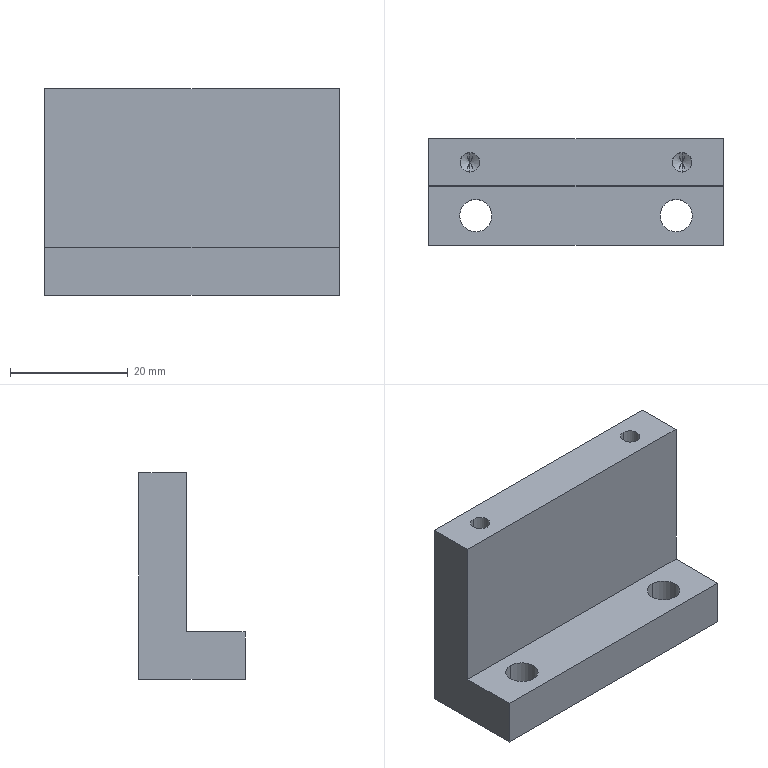Component | SolidWorks | LD101-02--Q1036-Q1-2-2 | 1 solid | 20 faces | box 50 x 18 x 35 mm | volume 17383 mm3 | cylinder 8 | plane 8 | cone 4 | commonest cylinder face diameters 5.5 x4 3.3 x4 | material AL6061
build123d program:
from build123d import *

# Parameters (mm, degrees)
SKETCH1_W             = 50
SKETCH1_H             = 35
BOSS_EXTRUDE1_DEPTH   = 9
SKETCH3_W             = 10
SKETCH3_H             = 27
CUT_EXTRUDE2_DEPTH    = 54.733
M4_TAPPED_HOLE1_D     = 3.3
M4_TAPPED_HOLE1_DEPTH = 13.5
M4_TAPPED_HOLE1_TIP   = 0.9914
SKETCH6_R             = 2.75
CUT_EXTRUDE3_DEPTH    = 38.881


with BuildPart() as part:
    # Sketch1 → Boss-Extrude1 (new, symmetric)
    with BuildSketch(Plane.XY):
        Rectangle(SKETCH1_W, SKETCH1_H)
    extrude(amount=BOSS_EXTRUDE1_DEPTH, both=True)

    # Sketch3 → Cut-Extrude2 (cut, through all)
    with BuildSketch(Plane.ZY.offset(25)):
        with Locations((4, 4)):
            Rectangle(SKETCH3_W, SKETCH3_H)
    extrude(amount=-CUT_EXTRUDE2_DEPTH, mode=Mode.SUBTRACT)

    # M4 Tapped Hole1
    with Locations(Plane(origin=(0, 17.5, 0), x_dir=(1, 0, 0), z_dir=(0, 1, 0))):
        with Locations((-18, 5), (18, 5)):
            Hole(M4_TAPPED_HOLE1_D / 2, depth=M4_TAPPED_HOLE1_DEPTH)
            with Locations((0, 0, -(M4_TAPPED_HOLE1_DEPTH + M4_TAPPED_HOLE1_TIP / 2))):  # 118° drill point
                Cone(0, M4_TAPPED_HOLE1_D / 2, M4_TAPPED_HOLE1_TIP, mode=Mode.SUBTRACT)

    # Sketch6 → Cut-Extrude3 (cut, through all)
    with BuildSketch(Plane(origin=(0, -9.5, 0), x_dir=(1, 0, 0), z_dir=(0, 1, 0))):
        with Locations(Location((-17, -4, 0), (0, 0, 270))):
            Circle(SKETCH6_R)
        with Locations(Location((17, -4, 0), (0, 0, 90))):
            Circle(SKETCH6_R)
    extrude(amount=-CUT_EXTRUDE3_DEPTH, mode=Mode.SUBTRACT)


solid = part.part

# Placed as in the assembly
solid = solid.moved(Location((121.71, -215.897, 310.757), (90, 0, 0)))
STEP:
#1=COLOUR_RGB('',0.7922,0.8196,0.9333);
#2=FILL_AREA_STYLE_COLOUR('',#1);
#3=FILL_AREA_STYLE('',(#2));
#4=SURFACE_STYLE_FILL_AREA(#3);
#5=SURFACE_SIDE_STYLE('',(#4));
#6=SURFACE_STYLE_USAGE(.BOTH.,#5);
#7=PRESENTATION_STYLE_ASSIGNMENT((#6));
#8=CARTESIAN_POINT('',(5.461,-8.549,11.546));
#9=VERTEX_POINT('',#8);
#10=CARTESIAN_POINT('',(5.461,-8.766,11.546));
#11=VERTEX_POINT('',#10);
#12=CARTESIAN_POINT('',(5.461,-8.657,11.546));
#13=DIRECTION('',(-0.,-0.,1.));
#14=DIRECTION('',(0.,1.,0.));
#15=AXIS2_PLACEMENT_3D('',#12,#13,#14);
#16=CIRCLE('',#15,0.1083);
#17=EDGE_CURVE('',#9,#11,#16,.T.);
#18=ORIENTED_EDGE('',*,*,#17,.F.);
#19=CARTESIAN_POINT('',(5.461,-8.549,11.86));
#20=VERTEX_POINT('',#19);
#21=CARTESIAN_POINT('',(5.461,-8.549,11.546));
#22=DIRECTION('',(-0.,-0.,1.));
#23=VECTOR('',#22,39.37);
#24=LINE('',#21,#23);
#25=EDGE_CURVE('',#9,#20,#24,.T.);
#26=ORIENTED_EDGE('',*,*,#25,.T.);
#27=CARTESIAN_POINT('',(5.461,-8.766,11.86));
#28=VERTEX_POINT('',#27);
#29=CARTESIAN_POINT('',(5.461,-8.657,11.86));
#30=DIRECTION('',(-0.,-0.,1.));
#31=DIRECTION('',(0.,1.,0.));
#32=AXIS2_PLACEMENT_3D('',#29,#30,#31);
#33=CIRCLE('',#32,0.1083);
#34=EDGE_CURVE('',#20,#28,#33,.T.);
#35=ORIENTED_EDGE('',*,*,#34,.T.);
#36=CARTESIAN_POINT('',(5.461,-8.766,11.546));
#37=DIRECTION('',(-0.,-0.,1.));
#38=VECTOR('',#37,39.37);
#39=LINE('',#36,#38);
#40=EDGE_CURVE('',#11,#28,#39,.T.);
#41=ORIENTED_EDGE('',*,*,#40,.F.);
#42=EDGE_LOOP('',(#18,#26,#35,#41));
#43=FACE_OUTER_BOUND('',#42,.T.);
#44=CARTESIAN_POINT('',(5.461,-8.657,11.546));
#45=DIRECTION('',(-0.,-0.,1.));
#46=DIRECTION('',(0.,-1.,0.));
#47=AXIS2_PLACEMENT_3D('',#44,#45,#46);
#48=CYLINDRICAL_SURFACE('',#47,0.1083);
#49=ADVANCED_FACE('',(#43),#48,.F.);
#50=CARTESIAN_POINT('',(4.122,-8.549,11.546));
#51=VERTEX_POINT('',#50);
#52=CARTESIAN_POINT('',(4.122,-8.766,11.546));
#53=VERTEX_POINT('',#52);
#54=CARTESIAN_POINT('',(4.122,-8.657,11.546));
#55=DIRECTION('',(-0.,-0.,1.));
#56=DIRECTION('',(0.,-1.,0.));
#57=AXIS2_PLACEMENT_3D('',#54,#55,#56);
#58=CIRCLE('',#57,0.1083);
#59=EDGE_CURVE('',#51,#53,#58,.T.);
#60=ORIENTED_EDGE('',*,*,#59,.F.);
#61=CARTESIAN_POINT('',(4.122,-8.549,11.86));
#62=VERTEX_POINT('',#61);
#63=CARTESIAN_POINT('',(4.122,-8.549,11.546));
#64=DIRECTION('',(-0.,-0.,1.));
#65=VECTOR('',#64,39.37);
#66=LINE('',#63,#65);
#67=EDGE_CURVE('',#51,#62,#66,.T.);
#68=ORIENTED_EDGE('',*,*,#67,.T.);
#69=CARTESIAN_POINT('',(4.122,-8.766,11.86));
#70=VERTEX_POINT('',#69);
#71=CARTESIAN_POINT('',(4.122,-8.657,11.86));
#72=DIRECTION('',(-0.,-0.,1.));
#73=DIRECTION('',(0.,-1.,0.));
#74=AXIS2_PLACEMENT_3D('',#71,#72,#73);
#75=CIRCLE('',#74,0.1083);
#76=EDGE_CURVE('',#62,#70,#75,.T.);
#77=ORIENTED_EDGE('',*,*,#76,.T.);
#78=CARTESIAN_POINT('',(4.122,-8.766,11.546));
#79=DIRECTION('',(-0.,-0.,1.));
#80=VECTOR('',#79,39.37);
#81=LINE('',#78,#80);
#82=EDGE_CURVE('',#53,#70,#81,.T.);
#83=ORIENTED_EDGE('',*,*,#82,.F.);
#84=EDGE_LOOP('',(#60,#68,#77,#83));
#85=FACE_OUTER_BOUND('',#84,.T.);
#86=CARTESIAN_POINT('',(4.122,-8.657,11.546));
#87=DIRECTION('',(-0.,-0.,1.));
#88=DIRECTION('',(0.,-1.,0.));
#89=AXIS2_PLACEMENT_3D('',#86,#87,#88);
#90=CYLINDRICAL_SURFACE('',#89,0.1083);
#91=ADVANCED_FACE('',(#85),#90,.F.);
#92=CARTESIAN_POINT('',(4.083,-8.238,12.392));
#93=VERTEX_POINT('',#92);
#94=CARTESIAN_POINT('',(4.083,-8.368,12.392));
#95=VERTEX_POINT('',#94);
#96=CARTESIAN_POINT('',(4.083,-8.303,12.392));
#97=DIRECTION('',(-0.,-0.,1.));
#98=DIRECTION('',(0.,-1.,0.));
#99=AXIS2_PLACEMENT_3D('',#96,#97,#98);
#100=CIRCLE('',#99,0.06496);
#101=EDGE_CURVE('',#93,#95,#100,.T.);
#102=ORIENTED_EDGE('',*,*,#101,.F.);
#103=CARTESIAN_POINT('',(4.083,-8.238,12.923));
#104=VERTEX_POINT('',#103);
#105=CARTESIAN_POINT('',(4.083,-8.238,12.923));
#106=DIRECTION('',(-0.,-0.,1.));
#107=VECTOR('',#106,39.37);
#108=LINE('',#105,#107);
#109=EDGE_CURVE('',#93,#104,#108,.T.);
#110=ORIENTED_EDGE('',*,*,#109,.T.);
#111=CARTESIAN_POINT('',(4.083,-8.368,12.923));
#112=VERTEX_POINT('',#111);
#113=CARTESIAN_POINT('',(4.083,-8.303,12.923));
#114=DIRECTION('',(-0.,-0.,1.));
#115=DIRECTION('',(0.,-1.,0.));
#116=AXIS2_PLACEMENT_3D('',#113,#114,#115);
#117=CIRCLE('',#116,0.06496);
#118=EDGE_CURVE('',#104,#112,#117,.T.);
#119=ORIENTED_EDGE('',*,*,#118,.T.);
#120=CARTESIAN_POINT('',(4.083,-8.368,12.923));
#121=DIRECTION('',(-0.,-0.,1.));
#122=VECTOR('',#121,39.37);
#123=LINE('',#120,#122);
#124=EDGE_CURVE('',#95,#112,#123,.T.);
#125=ORIENTED_EDGE('',*,*,#124,.F.);
#126=EDGE_LOOP('',(#102,#110,#119,#125));
#127=FACE_OUTER_BOUND('',#126,.T.);
#128=CARTESIAN_POINT('',(4.083,-8.303,12.923));
#129=DIRECTION('',(-0.,-0.,1.));
#130=DIRECTION('',(0.,-1.,0.));
#131=AXIS2_PLACEMENT_3D('',#128,#129,#130);
#132=CYLINDRICAL_SURFACE('',#131,0.06496);
#133=ADVANCED_FACE('',(#127),#132,.F.);
#134=CARTESIAN_POINT('',(4.083,-8.303,12.353));
#135=VERTEX_POINT('',#134);
#136=CARTESIAN_POINT('',(4.083,-8.368,12.392));
#137=DIRECTION('',(0.,-0.8572,0.515));
#138=VECTOR('',#137,39.37);
#139=LINE('',#136,#138);
#140=EDGE_CURVE('',#135,#95,#139,.T.);
#141=ORIENTED_EDGE('',*,*,#140,.F.);
#142=CARTESIAN_POINT('',(4.083,-8.238,12.392));
#143=DIRECTION('',(0.,0.8572,0.515));
#144=VECTOR('',#143,39.37);
#145=LINE('',#142,#144);
#146=EDGE_CURVE('',#135,#93,#145,.T.);
#147=ORIENTED_EDGE('',*,*,#146,.T.);
#148=ORIENTED_EDGE('',*,*,#101,.T.);
#149=EDGE_LOOP('',(#141,#147,#148));
#150=FACE_OUTER_BOUND('',#149,.T.);
#151=CARTESIAN_POINT('',(4.083,-8.303,12.392));
#152=DIRECTION('',(-0.,-0.,1.));
#153=DIRECTION('',(0.,-1.,0.));
#154=AXIS2_PLACEMENT_3D('',#151,#152,#153);
#155=CONICAL_SURFACE('',#154,0.06496,1.03);
#156=ADVANCED_FACE('',(#150),#155,.F.);
#157=CARTESIAN_POINT('',(5.5,-8.238,12.392));
#158=VERTEX_POINT('',#157);
#159=CARTESIAN_POINT('',(5.5,-8.368,12.392));
#160=VERTEX_POINT('',#159);
#161=CARTESIAN_POINT('',(5.5,-8.303,12.392));
#162=DIRECTION('',(-0.,-0.,1.));
#163=DIRECTION('',(0.,-1.,0.));
#164=AXIS2_PLACEMENT_3D('',#161,#162,#163);
#165=CIRCLE('',#164,0.06496);
#166=EDGE_CURVE('',#158,#160,#165,.T.);
#167=ORIENTED_EDGE('',*,*,#166,.F.);
#168=CARTESIAN_POINT('',(5.5,-8.238,12.923));
#169=VERTEX_POINT('',#168);
#170=CARTESIAN_POINT('',(5.5,-8.238,12.923));
#171=DIRECTION('',(-0.,-0.,1.));
#172=VECTOR('',#171,39.37);
#173=LINE('',#170,#172);
#174=EDGE_CURVE('',#158,#169,#173,.T.);
#175=ORIENTED_EDGE('',*,*,#174,.T.);
#176=CARTESIAN_POINT('',(5.5,-8.368,12.923));
#177=VERTEX_POINT('',#176);
#178=CARTESIAN_POINT('',(5.5,-8.303,12.923));
#179=DIRECTION('',(-0.,-0.,1.));
#180=DIRECTION('',(0.,-1.,0.));
#181=AXIS2_PLACEMENT_3D('',#178,#179,#180);
#182=CIRCLE('',#181,0.06496);
#183=EDGE_CURVE('',#169,#177,#182,.T.);
#184=ORIENTED_EDGE('',*,*,#183,.T.);
#185=CARTESIAN_POINT('',(5.5,-8.368,12.923));
#186=DIRECTION('',(-0.,-0.,1.));
#187=VECTOR('',#186,39.37);
#188=LINE('',#185,#187);
#189=EDGE_CURVE('',#160,#177,#188,.T.);
#190=ORIENTED_EDGE('',*,*,#189,.F.);
#191=EDGE_LOOP('',(#167,#175,#184,#190));
#192=FACE_OUTER_BOUND('',#191,.T.);
#193=CARTESIAN_POINT('',(5.5,-8.303,12.923));
#194=DIRECTION('',(-0.,-0.,1.));
#195=DIRECTION('',(0.,-1.,0.));
#196=AXIS2_PLACEMENT_3D('',#193,#194,#195);
#197=CYLINDRICAL_SURFACE('',#196,0.06496);
#198=ADVANCED_FACE('',(#192),#197,.F.);
#199=CARTESIAN_POINT('',(5.5,-8.303,12.353));
#200=VERTEX_POINT('',#199);
#201=CARTESIAN_POINT('',(5.5,-8.368,12.392));
#202=DIRECTION('',(0.,-0.8572,0.515));
#203=VECTOR('',#202,39.37);
#204=LINE('',#201,#203);
#205=EDGE_CURVE('',#200,#160,#204,.T.);
#206=ORIENTED_EDGE('',*,*,#205,.F.);
#207=CARTESIAN_POINT('',(5.5,-8.238,12.392));
#208=DIRECTION('',(0.,0.8572,0.515));
#209=VECTOR('',#208,39.37);
#210=LINE('',#207,#209);
#211=EDGE_CURVE('',#200,#158,#210,.T.);
#212=ORIENTED_EDGE('',*,*,#211,.T.);
#213=ORIENTED_EDGE('',*,*,#166,.T.);
#214=EDGE_LOOP('',(#206,#212,#213));
#215=FACE_OUTER_BOUND('',#214,.T.);
#216=CARTESIAN_POINT('',(5.5,-8.303,12.392));
#217=DIRECTION('',(-0.,-0.,1.));
#218=DIRECTION('',(0.,-1.,0.));
#219=AXIS2_PLACEMENT_3D('',#216,#217,#218);
#220=CONICAL_SURFACE('',#219,0.06496,1.03);
#221=ADVANCED_FACE('',(#215),#220,.F.);
#222=CARTESIAN_POINT('',(5.776,-8.461,12.923));
#223=VERTEX_POINT('',#222);
#224=CARTESIAN_POINT('',(5.776,-8.461,11.86));
#225=VERTEX_POINT('',#224);
#226=CARTESIAN_POINT('',(5.776,-8.461,12.923));
#227=DIRECTION('',(0.,-0.,-1.));
#228=VECTOR('',#227,39.37);
#229=LINE('',#226,#228);
#230=EDGE_CURVE('',#223,#225,#229,.T.);
#231=ORIENTED_EDGE('',*,*,#230,.T.);
#232=CARTESIAN_POINT('',(5.776,-8.854,11.86));
#233=VERTEX_POINT('',#232);
#234=CARTESIAN_POINT('',(5.776,-8.854,11.86));
#235=DIRECTION('',(0.,-1.,-0.));
#236=VECTOR('',#235,39.37);
#237=LINE('',#234,#236);
#238=EDGE_CURVE('',#225,#233,#237,.T.);
#239=ORIENTED_EDGE('',*,*,#238,.T.);
#240=CARTESIAN_POINT('',(5.776,-8.854,11.546));
#241=VERTEX_POINT('',#240);
#242=CARTESIAN_POINT('',(5.776,-8.854,11.546));
#243=DIRECTION('',(-0.,-0.,1.));
#244=VECTOR('',#243,39.37);
#245=LINE('',#242,#244);
#246=EDGE_CURVE('',#241,#233,#245,.T.);
#247=ORIENTED_EDGE('',*,*,#246,.F.);
#248=CARTESIAN_POINT('',(5.776,-8.146,11.546));
#249=VERTEX_POINT('',#248);
#250=CARTESIAN_POINT('',(5.776,-8.854,11.546));
#251=DIRECTION('',(-0.,1.,0.));
#252=VECTOR('',#251,39.37);
#253=LINE('',#250,#252);
#254=EDGE_CURVE('',#241,#249,#253,.T.);
#255=ORIENTED_EDGE('',*,*,#254,.T.);
#256=CARTESIAN_POINT('',(5.776,-8.146,12.923));
#257=VERTEX_POINT('',#256);
#258=CARTESIAN_POINT('',(5.776,-8.146,11.546));
#259=DIRECTION('',(-0.,-0.,1.));
#260=VECTOR('',#259,39.37);
#261=LINE('',#258,#260);
#262=EDGE_CURVE('',#249,#257,#261,.T.);
#263=ORIENTED_EDGE('',*,*,#262,.T.);
#264=CARTESIAN_POINT('',(5.776,-8.854,12.923));
#265=DIRECTION('',(-0.,1.,0.));
#266=VECTOR('',#265,39.37);
#267=LINE('',#264,#266);
#268=EDGE_CURVE('',#223,#257,#267,.T.);
#269=ORIENTED_EDGE('',*,*,#268,.F.);
#270=EDGE_LOOP('',(#231,#239,#247,#255,#263,#269));
#271=FACE_OUTER_BOUND('',#270,.T.);
#272=CARTESIAN_POINT('',(5.776,-8.854,11.546));
#273=DIRECTION('',(-1.,-0.,-0.));
#274=DIRECTION('',(0.,-1.,-0.));
#275=AXIS2_PLACEMENT_3D('',#272,#273,#274);
#276=PLANE('',#275);
#277=ADVANCED_FACE('',(#271),#276,.F.);
#278=CARTESIAN_POINT('',(4.083,-8.303,12.923));
#279=DIRECTION('',(-0.,-0.,1.));
#280=DIRECTION('',(0.,-1.,0.));
#281=AXIS2_PLACEMENT_3D('',#278,#279,#280);
#282=CIRCLE('',#281,0.06496);
#283=EDGE_CURVE('',#112,#104,#282,.T.);
#284=ORIENTED_EDGE('',*,*,#283,.F.);
#285=ORIENTED_EDGE('',*,*,#118,.F.);
#286=EDGE_LOOP('',(#284,#285));
#287=FACE_BOUND('',#286,.T.);
#288=CARTESIAN_POINT('',(5.5,-8.303,12.923));
#289=DIRECTION('',(-0.,-0.,1.));
#290=DIRECTION('',(0.,-1.,0.));
#291=AXIS2_PLACEMENT_3D('',#288,#289,#290);
#292=CIRCLE('',#291,0.06496);
#293=EDGE_CURVE('',#177,#169,#292,.T.);
#294=ORIENTED_EDGE('',*,*,#293,.F.);
#295=ORIENTED_EDGE('',*,*,#183,.F.);
#296=EDGE_LOOP('',(#294,#295));
#297=FACE_BOUND('',#296,.T.);
#298=CARTESIAN_POINT('',(3.807,-8.461,12.923));
#299=VERTEX_POINT('',#298);
#300=CARTESIAN_POINT('',(3.807,-8.146,12.923));
#301=VERTEX_POINT('',#300);
#302=CARTESIAN_POINT('',(3.807,-8.854,12.923));
#303=DIRECTION('',(-0.,1.,0.));
#304=VECTOR('',#303,39.37);
#305=LINE('',#302,#304);
#306=EDGE_CURVE('',#299,#301,#305,.T.);
#307=ORIENTED_EDGE('',*,*,#306,.F.);
#308=CARTESIAN_POINT('',(5.776,-8.461,12.923));
#309=DIRECTION('',(-1.,-0.,-0.));
#310=VECTOR('',#309,39.37);
#311=LINE('',#308,#310);
#312=EDGE_CURVE('',#223,#299,#311,.T.);
#313=ORIENTED_EDGE('',*,*,#312,.F.);
#314=ORIENTED_EDGE('',*,*,#268,.T.);
#315=CARTESIAN_POINT('',(3.807,-8.146,12.923));
#316=DIRECTION('',(-1.,-0.,-0.));
#317=VECTOR('',#316,39.37);
#318=LINE('',#315,#317);
#319=EDGE_CURVE('',#257,#301,#318,.T.);
#320=ORIENTED_EDGE('',*,*,#319,.T.);
#321=EDGE_LOOP('',(#307,#313,#314,#320));
#322=FACE_OUTER_BOUND('',#321,.T.);
#323=CARTESIAN_POINT('',(3.807,-8.854,12.923));
#324=DIRECTION('',(0.,0.,-1.));
#325=DIRECTION('',(-0.,1.,0.));
#326=AXIS2_PLACEMENT_3D('',#323,#324,#325);
#327=PLANE('',#326);
#328=ADVANCED_FACE('',(#287,#297,#322),#327,.F.);
#329=CARTESIAN_POINT('',(3.807,-8.854,11.86));
#330=VERTEX_POINT('',#329);
#331=CARTESIAN_POINT('',(3.807,-8.854,11.546));
#332=VERTEX_POINT('',#331);
#333=CARTESIAN_POINT('',(3.807,-8.854,11.546));
#334=DIRECTION('',(0.,0.,-1.));
#335=VECTOR('',#334,39.37);
#336=LINE('',#333,#335);
#337=EDGE_CURVE('',#330,#332,#336,.T.);
#338=ORIENTED_EDGE('',*,*,#337,.F.);
#339=CARTESIAN_POINT('',(3.807,-8.461,11.86));
#340=VERTEX_POINT('',#339);
#341=CARTESIAN_POINT('',(3.807,-8.854,11.86));
#342=DIRECTION('',(0.,-1.,-0.));
#343=VECTOR('',#342,39.37);
#344=LINE('',#341,#343);
#345=EDGE_CURVE('',#340,#330,#344,.T.);
#346=ORIENTED_EDGE('',*,*,#345,.F.);
#347=CARTESIAN_POINT('',(3.807,-8.461,12.923));
#348=DIRECTION('',(0.,-0.,-1.));
#349=VECTOR('',#348,39.37);
#350=LINE('',#347,#349);
#351=EDGE_CURVE('',#299,#340,#350,.T.);
#352=ORIENTED_EDGE('',*,*,#351,.F.);
#353=ORIENTED_EDGE('',*,*,#306,.T.);
#354=CARTESIAN_POINT('',(3.807,-8.146,11.546));
#355=VERTEX_POINT('',#354);
#356=CARTESIAN_POINT('',(3.807,-8.146,11.546));
#357=DIRECTION('',(0.,0.,-1.));
#358=VECTOR('',#357,39.37);
#359=LINE('',#356,#358);
#360=EDGE_CURVE('',#301,#355,#359,.T.);
#361=ORIENTED_EDGE('',*,*,#360,.T.);
#362=CARTESIAN_POINT('',(3.807,-8.854,11.546));
#363=DIRECTION('',(-0.,1.,0.));
#364=VECTOR('',#363,39.37);
#365=LINE('',#362,#364);
#366=EDGE_CURVE('',#332,#355,#365,.T.);
#367=ORIENTED_EDGE('',*,*,#366,.F.);
#368=EDGE_LOOP('',(#338,#346,#352,#353,#361,#367));
#369=FACE_OUTER_BOUND('',#368,.T.);
#370=CARTESIAN_POINT('',(3.807,-8.854,11.546));
#371=DIRECTION('',(1.,0.,0.));
#372=DIRECTION('',(-0.,1.,0.));
#373=AXIS2_PLACEMENT_3D('',#370,#371,#372);
#374=PLANE('',#373);
#375=ADVANCED_FACE('',(#369),#374,.F.);
#376=CARTESIAN_POINT('',(5.461,-8.657,11.546));
#377=DIRECTION('',(-0.,-0.,1.));
#378=DIRECTION('',(0.,1.,0.));
#379=AXIS2_PLACEMENT_3D('',#376,#377,#378);
#380=CIRCLE('',#379,0.1083);
#381=EDGE_CURVE('',#11,#9,#380,.T.);
#382=ORIENTED_EDGE('',*,*,#381,.T.);
#383=ORIENTED_EDGE('',*,*,#17,.T.);
#384=EDGE_LOOP('',(#382,#383));
#385=FACE_BOUND('',#384,.T.);
#386=CARTESIAN_POINT('',(4.122,-8.657,11.546));
#387=DIRECTION('',(-0.,-0.,1.));
#388=DIRECTION('',(0.,-1.,0.));
#389=AXIS2_PLACEMENT_3D('',#386,#387,#388);
#390=CIRCLE('',#389,0.1083);
#391=EDGE_CURVE('',#53,#51,#390,.T.);
#392=ORIENTED_EDGE('',*,*,#391,.T.);
#393=ORIENTED_EDGE('',*,*,#59,.T.);
#394=EDGE_LOOP('',(#392,#393));
#395=FACE_BOUND('',#394,.T.);
#396=CARTESIAN_POINT('',(3.807,-8.146,11.546));
#397=DIRECTION('',(1.,0.,0.));
#398=VECTOR('',#397,39.37);
#399=LINE('',#396,#398);
#400=EDGE_CURVE('',#355,#249,#399,.T.);
#401=ORIENTED_EDGE('',*,*,#400,.T.);
#402=ORIENTED_EDGE('',*,*,#254,.F.);
#403=CARTESIAN_POINT('',(3.807,-8.854,11.546));
#404=DIRECTION('',(1.,0.,0.));
#405=VECTOR('',#404,39.37);
#406=LINE('',#403,#405);
#407=EDGE_CURVE('',#332,#241,#406,.T.);
#408=ORIENTED_EDGE('',*,*,#407,.F.);
#409=ORIENTED_EDGE('',*,*,#366,.T.);
#410=EDGE_LOOP('',(#401,#402,#408,#409));
#411=FACE_OUTER_BOUND('',#410,.T.);
#412=CARTESIAN_POINT('',(3.807,-8.854,11.546));
#413=DIRECTION('',(-0.,-0.,1.));
#414=DIRECTION('',(0.,-1.,-0.));
#415=AXIS2_PLACEMENT_3D('',#412,#413,#414);
#416=PLANE('',#415);
#417=ADVANCED_FACE('',(#385,#395,#411),#416,.F.);
#418=ORIENTED_EDGE('',*,*,#246,.T.);
#419=CARTESIAN_POINT('',(5.776,-8.854,11.86));
#420=DIRECTION('',(-1.,-0.,-0.));
#421=VECTOR('',#420,39.37);
#422=LINE('',#419,#421);
#423=EDGE_CURVE('',#233,#330,#422,.T.);
#424=ORIENTED_EDGE('',*,*,#423,.T.);
#425=ORIENTED_EDGE('',*,*,#337,.T.);
#426=ORIENTED_EDGE('',*,*,#407,.T.);
#427=EDGE_LOOP('',(#418,#424,#425,#426));
#428=FACE_OUTER_BOUND('',#427,.T.);
#429=CARTESIAN_POINT('',(4.792,-8.854,12.235));
#430=DIRECTION('',(-0.,1.,0.));
#431=DIRECTION('',(-1.,-0.,-0.));
#432=AXIS2_PLACEMENT_3D('',#429,#430,#431);
#433=PLANE('',#432);
#434=ADVANCED_FACE('',(#428),#433,.F.);
#435=ORIENTED_EDGE('',*,*,#262,.F.);
#436=ORIENTED_EDGE('',*,*,#400,.F.);
#437=ORIENTED_EDGE('',*,*,#360,.F.);
#438=ORIENTED_EDGE('',*,*,#319,.F.);
#439=EDGE_LOOP('',(#435,#436,#437,#438));
#440=FACE_OUTER_BOUND('',#439,.T.);
#441=CARTESIAN_POINT('',(4.792,-8.146,12.235));
#442=DIRECTION('',(-0.,1.,0.));
#443=DIRECTION('',(-1.,-0.,-0.));
#444=AXIS2_PLACEMENT_3D('',#441,#442,#443);
#445=PLANE('',#444);
#446=ADVANCED_FACE('',(#440),#445,.T.);
#447=CARTESIAN_POINT('',(5.461,-8.657,11.86));
#448=DIRECTION('',(-0.,-0.,1.));
#449=DIRECTION('',(0.,1.,0.));
#450=AXIS2_PLACEMENT_3D('',#447,#448,#449);
#451=CIRCLE('',#450,0.1083);
#452=EDGE_CURVE('',#28,#20,#451,.T.);
#453=ORIENTED_EDGE('',*,*,#452,.F.);
#454=ORIENTED_EDGE('',*,*,#34,.F.);
#455=EDGE_LOOP('',(#453,#454));
#456=FACE_BOUND('',#455,.T.);
#457=CARTESIAN_POINT('',(4.122,-8.657,11.86));
#458=DIRECTION('',(-0.,-0.,1.));
#459=DIRECTION('',(0.,-1.,0.));
#460=AXIS2_PLACEMENT_3D('',#457,#458,#459);
#461=CIRCLE('',#460,0.1083);
#462=EDGE_CURVE('',#70,#62,#461,.T.);
#463=ORIENTED_EDGE('',*,*,#462,.F.);
#464=ORIENTED_EDGE('',*,*,#76,.F.);
#465=EDGE_LOOP('',(#463,#464));
#466=FACE_BOUND('',#465,.T.);
#467=ORIENTED_EDGE('',*,*,#345,.T.);
#468=ORIENTED_EDGE('',*,*,#423,.F.);
#469=ORIENTED_EDGE('',*,*,#238,.F.);
#470=CARTESIAN_POINT('',(5.776,-8.461,11.86));
#471=DIRECTION('',(-1.,-0.,-0.));
#472=VECTOR('',#471,39.37);
#473=LINE('',#470,#472);
#474=EDGE_CURVE('',#225,#340,#473,.T.);
#475=ORIENTED_EDGE('',*,*,#474,.T.);
#476=EDGE_LOOP('',(#467,#468,#469,#475));
#477=FACE_OUTER_BOUND('',#476,.T.);
#478=CARTESIAN_POINT('',(5.776,-8.854,11.86));
#479=DIRECTION('',(0.,0.,-1.));
#480=DIRECTION('',(-0.,1.,0.));
#481=AXIS2_PLACEMENT_3D('',#478,#479,#480);
#482=PLANE('',#481);
#483=ADVANCED_FACE('',(#456,#466,#477),#482,.F.);
#484=ORIENTED_EDGE('',*,*,#351,.T.);
#485=ORIENTED_EDGE('',*,*,#474,.F.);
#486=ORIENTED_EDGE('',*,*,#230,.F.);
#487=ORIENTED_EDGE('',*,*,#312,.T.);
#488=EDGE_LOOP('',(#484,#485,#486,#487));
#489=FACE_OUTER_BOUND('',#488,.T.);
#490=CARTESIAN_POINT('',(5.776,-8.461,12.923));
#491=DIRECTION('',(-0.,1.,-0.));
#492=DIRECTION('',(-0.,0.,1.));
#493=AXIS2_PLACEMENT_3D('',#490,#491,#492);
#494=PLANE('',#493);
#495=ADVANCED_FACE('',(#489),#494,.F.);
#496=ORIENTED_EDGE('',*,*,#211,.F.);
#497=ORIENTED_EDGE('',*,*,#205,.T.);
#498=CARTESIAN_POINT('',(5.5,-8.303,12.392));
#499=DIRECTION('',(-0.,-0.,1.));
#500=DIRECTION('',(0.,-1.,0.));
#501=AXIS2_PLACEMENT_3D('',#498,#499,#500);
#502=CIRCLE('',#501,0.06496);
#503=EDGE_CURVE('',#160,#158,#502,.T.);
#504=ORIENTED_EDGE('',*,*,#503,.T.);
#505=EDGE_LOOP('',(#496,#497,#504));
#506=FACE_OUTER_BOUND('',#505,.T.);
#507=CARTESIAN_POINT('',(5.5,-8.303,12.392));
#508=DIRECTION('',(-0.,-0.,1.));
#509=DIRECTION('',(0.,-1.,0.));
#510=AXIS2_PLACEMENT_3D('',#507,#508,#509);
#511=CONICAL_SURFACE('',#510,0.06496,1.03);
#512=ADVANCED_FACE('',(#506),#511,.F.);
#513=ORIENTED_EDGE('',*,*,#174,.F.);
#514=ORIENTED_EDGE('',*,*,#503,.F.);
#515=ORIENTED_EDGE('',*,*,#189,.T.);
#516=ORIENTED_EDGE('',*,*,#293,.T.);
#517=EDGE_LOOP('',(#513,#514,#515,#516));
#518=FACE_OUTER_BOUND('',#517,.T.);
#519=CARTESIAN_POINT('',(5.5,-8.303,12.923));
#520=DIRECTION('',(-0.,-0.,1.));
#521=DIRECTION('',(0.,-1.,0.));
#522=AXIS2_PLACEMENT_3D('',#519,#520,#521);
#523=CYLINDRICAL_SURFACE('',#522,0.06496);
#524=ADVANCED_FACE('',(#518),#523,.F.);
#525=ORIENTED_EDGE('',*,*,#146,.F.);
#526=ORIENTED_EDGE('',*,*,#140,.T.);
#527=CARTESIAN_POINT('',(4.083,-8.303,12.392));
#528=DIRECTION('',(-0.,-0.,1.));
#529=DIRECTION('',(0.,-1.,0.));
#530=AXIS2_PLACEMENT_3D('',#527,#528,#529);
#531=CIRCLE('',#530,0.06496);
#532=EDGE_CURVE('',#95,#93,#531,.T.);
#533=ORIENTED_EDGE('',*,*,#532,.T.);
#534=EDGE_LOOP('',(#525,#526,#533));
#535=FACE_OUTER_BOUND('',#534,.T.);
#536=CARTESIAN_POINT('',(4.083,-8.303,12.392));
#537=DIRECTION('',(-0.,-0.,1.));
#538=DIRECTION('',(0.,-1.,0.));
#539=AXIS2_PLACEMENT_3D('',#536,#537,#538);
#540=CONICAL_SURFACE('',#539,0.06496,1.03);
#541=ADVANCED_FACE('',(#535),#540,.F.);
#542=ORIENTED_EDGE('',*,*,#109,.F.);
#543=ORIENTED_EDGE('',*,*,#532,.F.);
#544=ORIENTED_EDGE('',*,*,#124,.T.);
#545=ORIENTED_EDGE('',*,*,#283,.T.);
#546=EDGE_LOOP('',(#542,#543,#544,#545));
#547=FACE_OUTER_BOUND('',#546,.T.);
#548=CARTESIAN_POINT('',(4.083,-8.303,12.923));
#549=DIRECTION('',(-0.,-0.,1.));
#550=DIRECTION('',(0.,-1.,0.));
#551=AXIS2_PLACEMENT_3D('',#548,#549,#550);
#552=CYLINDRICAL_SURFACE('',#551,0.06496);
#553=ADVANCED_FACE('',(#547),#552,.F.);
#554=ORIENTED_EDGE('',*,*,#67,.F.);
#555=ORIENTED_EDGE('',*,*,#391,.F.);
#556=ORIENTED_EDGE('',*,*,#82,.T.);
#557=ORIENTED_EDGE('',*,*,#462,.T.);
#558=EDGE_LOOP('',(#554,#555,#556,#557));
#559=FACE_OUTER_BOUND('',#558,.T.);
#560=CARTESIAN_POINT('',(4.122,-8.657,11.546));
#561=DIRECTION('',(-0.,-0.,1.));
#562=DIRECTION('',(0.,-1.,0.));
#563=AXIS2_PLACEMENT_3D('',#560,#561,#562);
#564=CYLINDRICAL_SURFACE('',#563,0.1083);
#565=ADVANCED_FACE('',(#559),#564,.F.);
#566=ORIENTED_EDGE('',*,*,#25,.F.);
#567=ORIENTED_EDGE('',*,*,#381,.F.);
#568=ORIENTED_EDGE('',*,*,#40,.T.);
#569=ORIENTED_EDGE('',*,*,#452,.T.);
#570=EDGE_LOOP('',(#566,#567,#568,#569));
#571=FACE_OUTER_BOUND('',#570,.T.);
#572=CARTESIAN_POINT('',(5.461,-8.657,11.546));
#573=DIRECTION('',(-0.,-0.,1.));
#574=DIRECTION('',(0.,-1.,0.));
#575=AXIS2_PLACEMENT_3D('',#572,#573,#574);
#576=CYLINDRICAL_SURFACE('',#575,0.1083);
#577=ADVANCED_FACE('',(#571),#576,.F.);
#578=CLOSED_SHELL('',(#49,#91,#133,#156,#198,#221,#277,#328,#375,#417,#434,#446,#483,#495,#512,#524,#541,#553,#565,#577));
#579=MANIFOLD_SOLID_BREP('',#578);
#580=STYLED_ITEM('',(#7),#579);
#581=(LENGTH_UNIT()NAMED_UNIT(*)SI_UNIT($,.METRE.));
#582=LENGTH_MEASURE_WITH_UNIT(LENGTH_MEASURE(0.0254),#581);
#583=DIMENSIONAL_EXPONENTS(1.,0.,0.,0.,0.,0.,0.);
#584=(CONVERSION_BASED_UNIT('',#582)LENGTH_UNIT()NAMED_UNIT(#583));
#585=UNCERTAINTY_MEASURE_WITH_UNIT(LENGTH_MEASURE(0.00001),#584,'','');
#586=(NAMED_UNIT(*)PLANE_ANGLE_UNIT()SI_UNIT($,.RADIAN.));
#587=(NAMED_UNIT(*)SI_UNIT($,.STERADIAN.)SOLID_ANGLE_UNIT());
#588=(GEOMETRIC_REPRESENTATION_CONTEXT(3)GLOBAL_UNCERTAINTY_ASSIGNED_CONTEXT((#585))GLOBAL_UNIT_ASSIGNED_CONTEXT((#584,#586,#587))REPRESENTATION_CONTEXT('',''));
#589=MECHANICAL_DESIGN_GEOMETRIC_PRESENTATION_REPRESENTATION('',(#580),#588);
#590=CARTESIAN_POINT('',(0.,0.,0.));
#591=DIRECTION('',(0.,0.,1.));
#592=DIRECTION('',(1.,0.,0.));
#593=AXIS2_PLACEMENT_3D('',#590,#591,#592);
#594=(LENGTH_UNIT()NAMED_UNIT(*)SI_UNIT($,.METRE.));
#595=LENGTH_MEASURE_WITH_UNIT(LENGTH_MEASURE(0.0254),#594);
#596=DIMENSIONAL_EXPONENTS(1.,0.,0.,0.,0.,0.,0.);
#597=(CONVERSION_BASED_UNIT('',#595)LENGTH_UNIT()NAMED_UNIT(#596));
#598=UNCERTAINTY_MEASURE_WITH_UNIT(LENGTH_MEASURE(0.00001),#597,'','');
#599=(NAMED_UNIT(*)PLANE_ANGLE_UNIT()SI_UNIT($,.RADIAN.));
#600=(NAMED_UNIT(*)SI_UNIT($,.STERADIAN.)SOLID_ANGLE_UNIT());
#601=(GEOMETRIC_REPRESENTATION_CONTEXT(3)GLOBAL_UNCERTAINTY_ASSIGNED_CONTEXT((#598))GLOBAL_UNIT_ASSIGNED_CONTEXT((#597,#599,#600))REPRESENTATION_CONTEXT('',''));
#602=ADVANCED_BREP_SHAPE_REPRESENTATION('',(#579,#593),#601);
#603=PRESENTATION_LAYER_ASSIGNMENT('','',(#580));